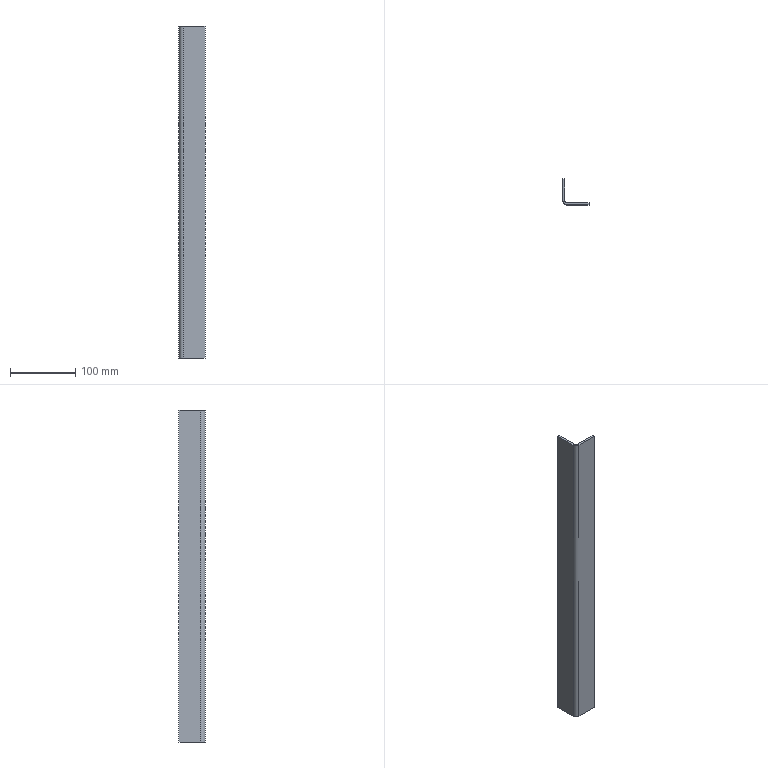Component | SolidWorks | BoxWelding-1_Beam1.1-1 | 1 solid | 10 faces | box 40 x 40 x 510 mm | volume 114527 mm3 | plane 8 | cylinder 2 | commonest cylinder face diameters 7 x1 13 x1
build123d program:
from build123d import *

# Parameters (mm, degrees)
EXTRUDE_THIN1_DEPTH = 255


with BuildPart() as part:
    # Sketch1 → Extrude-Thin1 (new, symmetric)
    with BuildSketch(Plane.XY):
        with BuildLine():
            Line((-1.5, 38.5), (-1.5, 5))
            ThreePointArc((-1.5, 5), (0.4038, 0.4038), (5, -1.5))
            Line((5, -1.5), (38.5, -1.5))
            Line((38.5, -1.5), (38.5, 1.5))
            Line((38.5, 1.5), (5, 1.5))
            ThreePointArc((5, 1.5), (2.525, 2.525), (1.5, 5))
            Line((1.5, 5), (1.5, 38.5))
            Line((1.5, 38.5), (-1.5, 38.5))
        make_face()
    extrude(amount=EXTRUDE_THIN1_DEPTH, both=True)


solid = part.part

# Placed as in the assembly
solid = solid.moved(Location((58.122, 788.001, 100.013), (0, 0, 0)))
STEP:
#1=COLOUR_RGB('',0.7922,0.8196,0.9333);
#2=FILL_AREA_STYLE_COLOUR('',#1);
#3=FILL_AREA_STYLE('',(#2));
#4=SURFACE_STYLE_FILL_AREA(#3);
#5=SURFACE_SIDE_STYLE('',(#4));
#6=SURFACE_STYLE_USAGE(.BOTH.,#5);
#7=PRESENTATION_STYLE_ASSIGNMENT((#6));
#8=CARTESIAN_POINT('',(2.485,30.965,-6.102));
#9=VERTEX_POINT('',#8);
#10=CARTESIAN_POINT('',(3.804,30.965,-6.102));
#11=VERTEX_POINT('',#10);
#12=CARTESIAN_POINT('',(2.485,30.965,-6.102));
#13=DIRECTION('',(1.,0.,0.));
#14=VECTOR('',#13,39.37);
#15=LINE('',#12,#14);
#16=EDGE_CURVE('',#9,#11,#15,.T.);
#17=ORIENTED_EDGE('',*,*,#16,.T.);
#18=CARTESIAN_POINT('',(3.804,30.965,13.977));
#19=VERTEX_POINT('',#18);
#20=CARTESIAN_POINT('',(3.804,30.965,13.977));
#21=DIRECTION('',(0.,0.,-1.));
#22=VECTOR('',#21,39.37);
#23=LINE('',#20,#22);
#24=EDGE_CURVE('',#19,#11,#23,.T.);
#25=ORIENTED_EDGE('',*,*,#24,.F.);
#26=CARTESIAN_POINT('',(2.485,30.965,13.977));
#27=VERTEX_POINT('',#26);
#28=CARTESIAN_POINT('',(2.485,30.965,13.977));
#29=DIRECTION('',(1.,0.,0.));
#30=VECTOR('',#29,39.37);
#31=LINE('',#28,#30);
#32=EDGE_CURVE('',#27,#19,#31,.T.);
#33=ORIENTED_EDGE('',*,*,#32,.F.);
#34=CARTESIAN_POINT('',(2.485,30.965,13.977));
#35=DIRECTION('',(0.,0.,-1.));
#36=VECTOR('',#35,39.37);
#37=LINE('',#34,#36);
#38=EDGE_CURVE('',#27,#9,#37,.T.);
#39=ORIENTED_EDGE('',*,*,#38,.T.);
#40=EDGE_LOOP('',(#17,#25,#33,#39));
#41=FACE_OUTER_BOUND('',#40,.T.);
#42=CARTESIAN_POINT('',(2.485,30.965,13.977));
#43=DIRECTION('',(0.,1.,0.));
#44=DIRECTION('',(0.,0.,1.));
#45=AXIS2_PLACEMENT_3D('',#42,#43,#44);
#46=PLANE('',#45);
#47=ADVANCED_FACE('',(#41),#46,.F.);
#48=CARTESIAN_POINT('',(3.804,31.083,-6.102));
#49=VERTEX_POINT('',#48);
#50=CARTESIAN_POINT('',(3.804,31.083,-6.102));
#51=DIRECTION('',(0.,-1.,0.));
#52=VECTOR('',#51,39.37);
#53=LINE('',#50,#52);
#54=EDGE_CURVE('',#49,#11,#53,.T.);
#55=ORIENTED_EDGE('',*,*,#54,.F.);
#56=CARTESIAN_POINT('',(3.804,31.083,13.977));
#57=VERTEX_POINT('',#56);
#58=CARTESIAN_POINT('',(3.804,31.083,13.977));
#59=DIRECTION('',(0.,0.,-1.));
#60=VECTOR('',#59,39.37);
#61=LINE('',#58,#60);
#62=EDGE_CURVE('',#57,#49,#61,.T.);
#63=ORIENTED_EDGE('',*,*,#62,.F.);
#64=CARTESIAN_POINT('',(3.804,31.083,13.977));
#65=DIRECTION('',(0.,-1.,0.));
#66=VECTOR('',#65,39.37);
#67=LINE('',#64,#66);
#68=EDGE_CURVE('',#57,#19,#67,.T.);
#69=ORIENTED_EDGE('',*,*,#68,.T.);
#70=ORIENTED_EDGE('',*,*,#24,.T.);
#71=EDGE_LOOP('',(#55,#63,#69,#70));
#72=FACE_OUTER_BOUND('',#71,.T.);
#73=CARTESIAN_POINT('',(3.804,31.083,13.977));
#74=DIRECTION('',(1.,0.,0.));
#75=DIRECTION('',(0.,0.,-1.));
#76=AXIS2_PLACEMENT_3D('',#73,#74,#75);
#77=PLANE('',#76);
#78=ADVANCED_FACE('',(#72),#77,.T.);
#79=CARTESIAN_POINT('',(2.485,31.083,-6.102));
#80=VERTEX_POINT('',#79);
#81=CARTESIAN_POINT('',(2.485,31.083,-6.102));
#82=DIRECTION('',(1.,0.,0.));
#83=VECTOR('',#82,39.37);
#84=LINE('',#81,#83);
#85=EDGE_CURVE('',#80,#49,#84,.T.);
#86=ORIENTED_EDGE('',*,*,#85,.F.);
#87=CARTESIAN_POINT('',(2.485,31.083,13.977));
#88=VERTEX_POINT('',#87);
#89=CARTESIAN_POINT('',(2.485,31.083,13.977));
#90=DIRECTION('',(0.,0.,-1.));
#91=VECTOR('',#90,39.37);
#92=LINE('',#89,#91);
#93=EDGE_CURVE('',#88,#80,#92,.T.);
#94=ORIENTED_EDGE('',*,*,#93,.F.);
#95=CARTESIAN_POINT('',(2.485,31.083,13.977));
#96=DIRECTION('',(1.,0.,0.));
#97=VECTOR('',#96,39.37);
#98=LINE('',#95,#97);
#99=EDGE_CURVE('',#88,#57,#98,.T.);
#100=ORIENTED_EDGE('',*,*,#99,.T.);
#101=ORIENTED_EDGE('',*,*,#62,.T.);
#102=EDGE_LOOP('',(#86,#94,#100,#101));
#103=FACE_OUTER_BOUND('',#102,.T.);
#104=CARTESIAN_POINT('',(2.485,31.083,13.977));
#105=DIRECTION('',(0.,1.,0.));
#106=DIRECTION('',(0.,0.,1.));
#107=AXIS2_PLACEMENT_3D('',#104,#105,#106);
#108=PLANE('',#107);
#109=ADVANCED_FACE('',(#103),#108,.T.);
#110=CARTESIAN_POINT('',(2.347,31.221,-6.102));
#111=VERTEX_POINT('',#110);
#112=CARTESIAN_POINT('',(2.485,31.221,-6.102));
#113=DIRECTION('',(0.,0.,1.));
#114=DIRECTION('',(1.,0.,0.));
#115=AXIS2_PLACEMENT_3D('',#112,#113,#114);
#116=CIRCLE('',#115,0.1378);
#117=EDGE_CURVE('',#111,#80,#116,.T.);
#118=ORIENTED_EDGE('',*,*,#117,.F.);
#119=CARTESIAN_POINT('',(2.347,31.221,13.977));
#120=VERTEX_POINT('',#119);
#121=CARTESIAN_POINT('',(2.347,31.221,13.977));
#122=DIRECTION('',(0.,0.,-1.));
#123=VECTOR('',#122,39.37);
#124=LINE('',#121,#123);
#125=EDGE_CURVE('',#120,#111,#124,.T.);
#126=ORIENTED_EDGE('',*,*,#125,.F.);
#127=CARTESIAN_POINT('',(2.485,31.221,13.977));
#128=DIRECTION('',(0.,0.,1.));
#129=DIRECTION('',(1.,0.,0.));
#130=AXIS2_PLACEMENT_3D('',#127,#128,#129);
#131=CIRCLE('',#130,0.1378);
#132=EDGE_CURVE('',#120,#88,#131,.T.);
#133=ORIENTED_EDGE('',*,*,#132,.T.);
#134=ORIENTED_EDGE('',*,*,#93,.T.);
#135=EDGE_LOOP('',(#118,#126,#133,#134));
#136=FACE_OUTER_BOUND('',#135,.T.);
#137=CARTESIAN_POINT('',(2.485,31.221,13.977));
#138=DIRECTION('',(0.,0.,-1.));
#139=DIRECTION('',(-1.,0.,0.));
#140=AXIS2_PLACEMENT_3D('',#137,#138,#139);
#141=CYLINDRICAL_SURFACE('',#140,0.1378);
#142=ADVANCED_FACE('',(#136),#141,.F.);
#143=CARTESIAN_POINT('',(2.347,32.539,-6.102));
#144=VERTEX_POINT('',#143);
#145=CARTESIAN_POINT('',(2.347,32.539,-6.102));
#146=DIRECTION('',(-0.,-1.,0.));
#147=VECTOR('',#146,39.37);
#148=LINE('',#145,#147);
#149=EDGE_CURVE('',#144,#111,#148,.T.);
#150=ORIENTED_EDGE('',*,*,#149,.F.);
#151=CARTESIAN_POINT('',(2.347,32.539,13.977));
#152=VERTEX_POINT('',#151);
#153=CARTESIAN_POINT('',(2.347,32.539,13.977));
#154=DIRECTION('',(0.,0.,-1.));
#155=VECTOR('',#154,39.37);
#156=LINE('',#153,#155);
#157=EDGE_CURVE('',#152,#144,#156,.T.);
#158=ORIENTED_EDGE('',*,*,#157,.F.);
#159=CARTESIAN_POINT('',(2.347,32.539,13.977));
#160=DIRECTION('',(-0.,-1.,0.));
#161=VECTOR('',#160,39.37);
#162=LINE('',#159,#161);
#163=EDGE_CURVE('',#152,#120,#162,.T.);
#164=ORIENTED_EDGE('',*,*,#163,.T.);
#165=ORIENTED_EDGE('',*,*,#125,.T.);
#166=EDGE_LOOP('',(#150,#158,#164,#165));
#167=FACE_OUTER_BOUND('',#166,.T.);
#168=CARTESIAN_POINT('',(2.347,32.539,13.977));
#169=DIRECTION('',(1.,-0.,0.));
#170=DIRECTION('',(0.,1.,0.));
#171=AXIS2_PLACEMENT_3D('',#168,#169,#170);
#172=PLANE('',#171);
#173=ADVANCED_FACE('',(#167),#172,.T.);
#174=CARTESIAN_POINT('',(2.229,32.539,-6.102));
#175=VERTEX_POINT('',#174);
#176=CARTESIAN_POINT('',(2.229,32.539,-6.102));
#177=DIRECTION('',(1.,0.,0.));
#178=VECTOR('',#177,39.37);
#179=LINE('',#176,#178);
#180=EDGE_CURVE('',#175,#144,#179,.T.);
#181=ORIENTED_EDGE('',*,*,#180,.F.);
#182=CARTESIAN_POINT('',(2.229,32.539,13.977));
#183=VERTEX_POINT('',#182);
#184=CARTESIAN_POINT('',(2.229,32.539,13.977));
#185=DIRECTION('',(0.,0.,-1.));
#186=VECTOR('',#185,39.37);
#187=LINE('',#184,#186);
#188=EDGE_CURVE('',#183,#175,#187,.T.);
#189=ORIENTED_EDGE('',*,*,#188,.F.);
#190=CARTESIAN_POINT('',(2.229,32.539,13.977));
#191=DIRECTION('',(1.,0.,0.));
#192=VECTOR('',#191,39.37);
#193=LINE('',#190,#192);
#194=EDGE_CURVE('',#183,#152,#193,.T.);
#195=ORIENTED_EDGE('',*,*,#194,.T.);
#196=ORIENTED_EDGE('',*,*,#157,.T.);
#197=EDGE_LOOP('',(#181,#189,#195,#196));
#198=FACE_OUTER_BOUND('',#197,.T.);
#199=CARTESIAN_POINT('',(2.229,32.539,13.977));
#200=DIRECTION('',(0.,1.,0.));
#201=DIRECTION('',(0.,0.,1.));
#202=AXIS2_PLACEMENT_3D('',#199,#200,#201);
#203=PLANE('',#202);
#204=ADVANCED_FACE('',(#198),#203,.T.);
#205=CARTESIAN_POINT('',(2.229,31.221,-6.102));
#206=VERTEX_POINT('',#205);
#207=CARTESIAN_POINT('',(2.229,32.539,-6.102));
#208=DIRECTION('',(-0.,-1.,0.));
#209=VECTOR('',#208,39.37);
#210=LINE('',#207,#209);
#211=EDGE_CURVE('',#175,#206,#210,.T.);
#212=ORIENTED_EDGE('',*,*,#211,.T.);
#213=CARTESIAN_POINT('',(2.229,31.221,13.977));
#214=VERTEX_POINT('',#213);
#215=CARTESIAN_POINT('',(2.229,31.221,13.977));
#216=DIRECTION('',(0.,0.,-1.));
#217=VECTOR('',#216,39.37);
#218=LINE('',#215,#217);
#219=EDGE_CURVE('',#214,#206,#218,.T.);
#220=ORIENTED_EDGE('',*,*,#219,.F.);
#221=CARTESIAN_POINT('',(2.229,32.539,13.977));
#222=DIRECTION('',(-0.,-1.,0.));
#223=VECTOR('',#222,39.37);
#224=LINE('',#221,#223);
#225=EDGE_CURVE('',#183,#214,#224,.T.);
#226=ORIENTED_EDGE('',*,*,#225,.F.);
#227=ORIENTED_EDGE('',*,*,#188,.T.);
#228=EDGE_LOOP('',(#212,#220,#226,#227));
#229=FACE_OUTER_BOUND('',#228,.T.);
#230=CARTESIAN_POINT('',(2.229,32.539,13.977));
#231=DIRECTION('',(1.,-0.,0.));
#232=DIRECTION('',(0.,1.,0.));
#233=AXIS2_PLACEMENT_3D('',#230,#231,#232);
#234=PLANE('',#233);
#235=ADVANCED_FACE('',(#229),#234,.F.);
#236=CARTESIAN_POINT('',(2.485,31.221,-6.102));
#237=DIRECTION('',(0.,0.,1.));
#238=DIRECTION('',(1.,0.,0.));
#239=AXIS2_PLACEMENT_3D('',#236,#237,#238);
#240=CIRCLE('',#239,0.2559);
#241=EDGE_CURVE('',#206,#9,#240,.T.);
#242=ORIENTED_EDGE('',*,*,#241,.T.);
#243=ORIENTED_EDGE('',*,*,#38,.F.);
#244=CARTESIAN_POINT('',(2.485,31.221,13.977));
#245=DIRECTION('',(0.,0.,1.));
#246=DIRECTION('',(1.,0.,0.));
#247=AXIS2_PLACEMENT_3D('',#244,#245,#246);
#248=CIRCLE('',#247,0.2559);
#249=EDGE_CURVE('',#214,#27,#248,.T.);
#250=ORIENTED_EDGE('',*,*,#249,.F.);
#251=ORIENTED_EDGE('',*,*,#219,.T.);
#252=EDGE_LOOP('',(#242,#243,#250,#251));
#253=FACE_OUTER_BOUND('',#252,.T.);
#254=CARTESIAN_POINT('',(2.485,31.221,13.977));
#255=DIRECTION('',(0.,0.,-1.));
#256=DIRECTION('',(-1.,0.,0.));
#257=AXIS2_PLACEMENT_3D('',#254,#255,#256);
#258=CYLINDRICAL_SURFACE('',#257,0.2559);
#259=ADVANCED_FACE('',(#253),#258,.T.);
#260=ORIENTED_EDGE('',*,*,#32,.T.);
#261=ORIENTED_EDGE('',*,*,#68,.F.);
#262=ORIENTED_EDGE('',*,*,#99,.F.);
#263=ORIENTED_EDGE('',*,*,#132,.F.);
#264=ORIENTED_EDGE('',*,*,#163,.F.);
#265=ORIENTED_EDGE('',*,*,#194,.F.);
#266=ORIENTED_EDGE('',*,*,#225,.T.);
#267=ORIENTED_EDGE('',*,*,#249,.T.);
#268=EDGE_LOOP('',(#260,#261,#262,#263,#264,#265,#266,#267));
#269=FACE_OUTER_BOUND('',#268,.T.);
#270=CARTESIAN_POINT('',(2.485,31.221,13.977));
#271=DIRECTION('',(0.,0.,1.));
#272=DIRECTION('',(1.,0.,0.));
#273=AXIS2_PLACEMENT_3D('',#270,#271,#272);
#274=PLANE('',#273);
#275=ADVANCED_FACE('',(#269),#274,.T.);
#276=ORIENTED_EDGE('',*,*,#16,.F.);
#277=ORIENTED_EDGE('',*,*,#241,.F.);
#278=ORIENTED_EDGE('',*,*,#211,.F.);
#279=ORIENTED_EDGE('',*,*,#180,.T.);
#280=ORIENTED_EDGE('',*,*,#149,.T.);
#281=ORIENTED_EDGE('',*,*,#117,.T.);
#282=ORIENTED_EDGE('',*,*,#85,.T.);
#283=ORIENTED_EDGE('',*,*,#54,.T.);
#284=EDGE_LOOP('',(#276,#277,#278,#279,#280,#281,#282,#283));
#285=FACE_OUTER_BOUND('',#284,.T.);
#286=CARTESIAN_POINT('',(2.485,31.221,-6.102));
#287=DIRECTION('',(0.,0.,1.));
#288=DIRECTION('',(1.,0.,0.));
#289=AXIS2_PLACEMENT_3D('',#286,#287,#288);
#290=PLANE('',#289);
#291=ADVANCED_FACE('',(#285),#290,.F.);
#292=CLOSED_SHELL('',(#47,#78,#109,#142,#173,#204,#235,#259,#275,#291));
#293=MANIFOLD_SOLID_BREP('',#292);
#294=STYLED_ITEM('',(#7),#293);
#295=(LENGTH_UNIT()NAMED_UNIT(*)SI_UNIT($,.METRE.));
#296=LENGTH_MEASURE_WITH_UNIT(LENGTH_MEASURE(0.0254),#295);
#297=DIMENSIONAL_EXPONENTS(1.,0.,0.,0.,0.,0.,0.);
#298=(CONVERSION_BASED_UNIT('',#296)LENGTH_UNIT()NAMED_UNIT(#297));
#299=UNCERTAINTY_MEASURE_WITH_UNIT(LENGTH_MEASURE(0.00001),#298,'','');
#300=(NAMED_UNIT(*)PLANE_ANGLE_UNIT()SI_UNIT($,.RADIAN.));
#301=(NAMED_UNIT(*)SI_UNIT($,.STERADIAN.)SOLID_ANGLE_UNIT());
#302=(GEOMETRIC_REPRESENTATION_CONTEXT(3)GLOBAL_UNCERTAINTY_ASSIGNED_CONTEXT((#299))GLOBAL_UNIT_ASSIGNED_CONTEXT((#298,#300,#301))REPRESENTATION_CONTEXT('',''));
#303=MECHANICAL_DESIGN_GEOMETRIC_PRESENTATION_REPRESENTATION('',(#294),#302);
#304=PRESENTATION_LAYER_ASSIGNMENT('','',(#294));
#305=CARTESIAN_POINT('',(0.,0.,0.));
#306=DIRECTION('',(0.,0.,1.));
#307=DIRECTION('',(1.,0.,0.));
#308=AXIS2_PLACEMENT_3D('',#305,#306,#307);
#309=(LENGTH_UNIT()NAMED_UNIT(*)SI_UNIT($,.METRE.));
#310=LENGTH_MEASURE_WITH_UNIT(LENGTH_MEASURE(0.0254),#309);
#311=DIMENSIONAL_EXPONENTS(1.,0.,0.,0.,0.,0.,0.);
#312=(CONVERSION_BASED_UNIT('',#310)LENGTH_UNIT()NAMED_UNIT(#311));
#313=UNCERTAINTY_MEASURE_WITH_UNIT(LENGTH_MEASURE(0.00001),#312,'','');
#314=(NAMED_UNIT(*)PLANE_ANGLE_UNIT()SI_UNIT($,.RADIAN.));
#315=(NAMED_UNIT(*)SI_UNIT($,.STERADIAN.)SOLID_ANGLE_UNIT());
#316=(GEOMETRIC_REPRESENTATION_CONTEXT(3)GLOBAL_UNCERTAINTY_ASSIGNED_CONTEXT((#313))GLOBAL_UNIT_ASSIGNED_CONTEXT((#312,#314,#315))REPRESENTATION_CONTEXT('',''));
#317=ADVANCED_BREP_SHAPE_REPRESENTATION('',(#293,#308),#316);